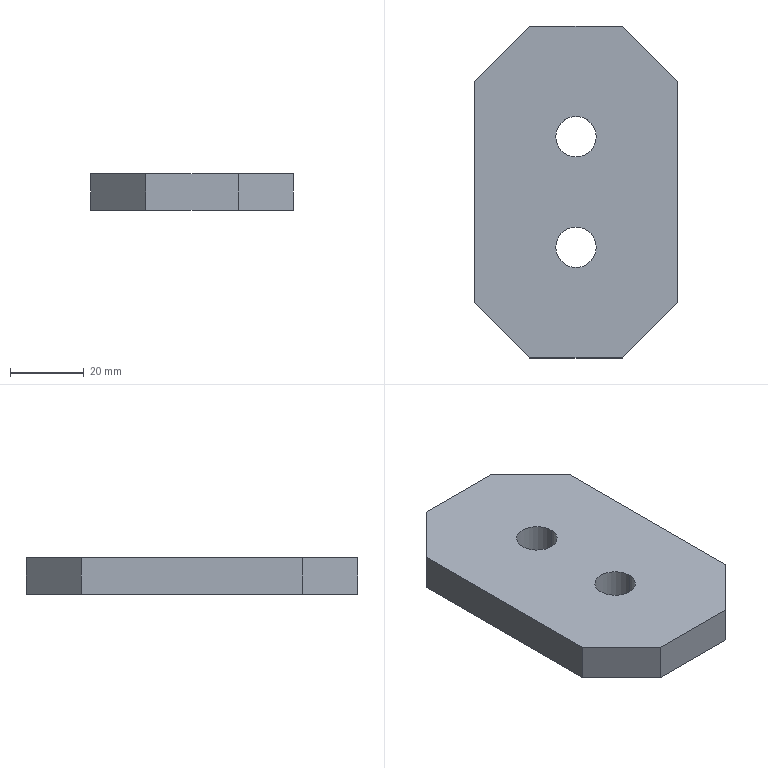Component | SolidWorks | 12ASlidingStraighteningWheelRetainingPlate-2 | 1 solid | 14 faces | box 55 x 90 x 10 mm | volume 43099 mm3 | plane 10 | cylinder 4 | commonest cylinder face diameters 11 x4 | material Q235
build123d program:
from build123d import *

# Parameters (mm, degrees)
BOSS_EXTRUDE1_DEPTH        = 10
F_11_0_11_DIAMETER_HOLE1_D = 11


with BuildPart() as part:
    # Sketch1 → Boss-Extrude1 (new body)
    with BuildSketch(Plane.XY):
        Polygon((-12.5, 45), (12.5, 45), (27.5, 30), (27.5, -30), (12.5, -45), (-12.5, -45), (-27.5, -30), (-27.5, 30), align=None)
    extrude(amount=BOSS_EXTRUDE1_DEPTH)

    # 11.0 _11_ Diameter Hole1 (through all)
    with Locations(Plane.XY.offset(10)):
        with Locations((0, -15), (0, 15)):
            Hole(F_11_0_11_DIAMETER_HOLE1_D / 2)


solid = part.part

# Placed as in the assembly
solid = solid.moved(Location((-213.402, 137.728, -24.25), (0, 0, 0)))
STEP:
#1=CARTESIAN_POINT('',(-8.185,6.013,-0.9547));
#2=VERTEX_POINT('',#1);
#3=CARTESIAN_POINT('',(-8.618,6.013,-0.9547));
#4=VERTEX_POINT('',#3);
#5=CARTESIAN_POINT('',(-8.402,6.013,-0.9547));
#6=DIRECTION('',(0.,0.,-1.));
#7=DIRECTION('',(-1.,0.,0.));
#8=AXIS2_PLACEMENT_3D('',#5,#6,#7);
#9=CIRCLE('',#8,0.2165);
#10=EDGE_CURVE('',#2,#4,#9,.T.);
#11=ORIENTED_EDGE('',*,*,#10,.T.);
#12=CARTESIAN_POINT('',(-8.618,6.013,-0.561));
#13=VERTEX_POINT('',#12);
#14=CARTESIAN_POINT('',(-8.618,6.013,-0.561));
#15=DIRECTION('',(0.,0.,1.));
#16=VECTOR('',#15,39.37);
#17=LINE('',#14,#16);
#18=EDGE_CURVE('',#4,#13,#17,.T.);
#19=ORIENTED_EDGE('',*,*,#18,.T.);
#20=CARTESIAN_POINT('',(-8.185,6.013,-0.561));
#21=VERTEX_POINT('',#20);
#22=CARTESIAN_POINT('',(-8.402,6.013,-0.561));
#23=DIRECTION('',(0.,0.,1.));
#24=DIRECTION('',(1.,0.,0.));
#25=AXIS2_PLACEMENT_3D('',#22,#23,#24);
#26=CIRCLE('',#25,0.2165);
#27=EDGE_CURVE('',#13,#21,#26,.T.);
#28=ORIENTED_EDGE('',*,*,#27,.T.);
#29=CARTESIAN_POINT('',(-8.185,6.013,-0.561));
#30=DIRECTION('',(0.,0.,1.));
#31=VECTOR('',#30,39.37);
#32=LINE('',#29,#31);
#33=EDGE_CURVE('',#2,#21,#32,.T.);
#34=ORIENTED_EDGE('',*,*,#33,.F.);
#35=EDGE_LOOP('',(#11,#19,#28,#34));
#36=FACE_OUTER_BOUND('',#35,.T.);
#37=CARTESIAN_POINT('',(-8.402,6.013,-0.561));
#38=DIRECTION('',(0.,0.,1.));
#39=DIRECTION('',(1.,0.,0.));
#40=AXIS2_PLACEMENT_3D('',#37,#38,#39);
#41=CYLINDRICAL_SURFACE('',#40,0.2165);
#42=ADVANCED_FACE('',(#36),#41,.F.);
#43=CARTESIAN_POINT('',(-8.185,4.832,-0.9547));
#44=VERTEX_POINT('',#43);
#45=CARTESIAN_POINT('',(-8.618,4.832,-0.9547));
#46=VERTEX_POINT('',#45);
#47=CARTESIAN_POINT('',(-8.402,4.832,-0.9547));
#48=DIRECTION('',(0.,0.,-1.));
#49=DIRECTION('',(-1.,0.,0.));
#50=AXIS2_PLACEMENT_3D('',#47,#48,#49);
#51=CIRCLE('',#50,0.2165);
#52=EDGE_CURVE('',#44,#46,#51,.T.);
#53=ORIENTED_EDGE('',*,*,#52,.T.);
#54=CARTESIAN_POINT('',(-8.618,4.832,-0.561));
#55=VERTEX_POINT('',#54);
#56=CARTESIAN_POINT('',(-8.618,4.832,-0.561));
#57=DIRECTION('',(0.,0.,1.));
#58=VECTOR('',#57,39.37);
#59=LINE('',#56,#58);
#60=EDGE_CURVE('',#46,#55,#59,.T.);
#61=ORIENTED_EDGE('',*,*,#60,.T.);
#62=CARTESIAN_POINT('',(-8.185,4.832,-0.561));
#63=VERTEX_POINT('',#62);
#64=CARTESIAN_POINT('',(-8.402,4.832,-0.561));
#65=DIRECTION('',(0.,0.,1.));
#66=DIRECTION('',(1.,0.,0.));
#67=AXIS2_PLACEMENT_3D('',#64,#65,#66);
#68=CIRCLE('',#67,0.2165);
#69=EDGE_CURVE('',#55,#63,#68,.T.);
#70=ORIENTED_EDGE('',*,*,#69,.T.);
#71=CARTESIAN_POINT('',(-8.185,4.832,-0.561));
#72=DIRECTION('',(0.,0.,1.));
#73=VECTOR('',#72,39.37);
#74=LINE('',#71,#73);
#75=EDGE_CURVE('',#44,#63,#74,.T.);
#76=ORIENTED_EDGE('',*,*,#75,.F.);
#77=EDGE_LOOP('',(#53,#61,#70,#76));
#78=FACE_OUTER_BOUND('',#77,.T.);
#79=CARTESIAN_POINT('',(-8.402,4.832,-0.561));
#80=DIRECTION('',(0.,0.,1.));
#81=DIRECTION('',(1.,0.,0.));
#82=AXIS2_PLACEMENT_3D('',#79,#80,#81);
#83=CYLINDRICAL_SURFACE('',#82,0.2165);
#84=ADVANCED_FACE('',(#78),#83,.F.);
#85=CARTESIAN_POINT('',(-8.402,4.832,-0.561));
#86=DIRECTION('',(0.,0.,1.));
#87=DIRECTION('',(1.,0.,0.));
#88=AXIS2_PLACEMENT_3D('',#85,#86,#87);
#89=CIRCLE('',#88,0.2165);
#90=EDGE_CURVE('',#63,#55,#89,.T.);
#91=ORIENTED_EDGE('',*,*,#90,.F.);
#92=ORIENTED_EDGE('',*,*,#69,.F.);
#93=EDGE_LOOP('',(#91,#92));
#94=FACE_BOUND('',#93,.T.);
#95=CARTESIAN_POINT('',(-8.894,7.194,-0.561));
#96=VERTEX_POINT('',#95);
#97=CARTESIAN_POINT('',(-9.484,6.603,-0.561));
#98=VERTEX_POINT('',#97);
#99=CARTESIAN_POINT('',(-9.484,6.603,-0.561));
#100=DIRECTION('',(-0.7071,-0.7071,0.));
#101=VECTOR('',#100,39.37);
#102=LINE('',#99,#101);
#103=EDGE_CURVE('',#96,#98,#102,.T.);
#104=ORIENTED_EDGE('',*,*,#103,.T.);
#105=CARTESIAN_POINT('',(-9.484,4.241,-0.561));
#106=VERTEX_POINT('',#105);
#107=CARTESIAN_POINT('',(-9.484,6.603,-0.561));
#108=DIRECTION('',(0.,-1.,0.));
#109=VECTOR('',#108,39.37);
#110=LINE('',#107,#109);
#111=EDGE_CURVE('',#98,#106,#110,.T.);
#112=ORIENTED_EDGE('',*,*,#111,.T.);
#113=CARTESIAN_POINT('',(-8.894,3.651,-0.561));
#114=VERTEX_POINT('',#113);
#115=CARTESIAN_POINT('',(-9.484,4.241,-0.561));
#116=DIRECTION('',(0.7071,-0.7071,0.));
#117=VECTOR('',#116,39.37);
#118=LINE('',#115,#117);
#119=EDGE_CURVE('',#106,#114,#118,.T.);
#120=ORIENTED_EDGE('',*,*,#119,.T.);
#121=CARTESIAN_POINT('',(-7.91,3.651,-0.561));
#122=VERTEX_POINT('',#121);
#123=CARTESIAN_POINT('',(-8.894,3.651,-0.561));
#124=DIRECTION('',(1.,0.,0.));
#125=VECTOR('',#124,39.37);
#126=LINE('',#123,#125);
#127=EDGE_CURVE('',#114,#122,#126,.T.);
#128=ORIENTED_EDGE('',*,*,#127,.T.);
#129=CARTESIAN_POINT('',(-7.319,4.241,-0.561));
#130=VERTEX_POINT('',#129);
#131=CARTESIAN_POINT('',(-7.319,4.241,-0.561));
#132=DIRECTION('',(0.7071,0.7071,0.));
#133=VECTOR('',#132,39.37);
#134=LINE('',#131,#133);
#135=EDGE_CURVE('',#122,#130,#134,.T.);
#136=ORIENTED_EDGE('',*,*,#135,.T.);
#137=CARTESIAN_POINT('',(-7.319,6.603,-0.561));
#138=VERTEX_POINT('',#137);
#139=CARTESIAN_POINT('',(-7.319,6.603,-0.561));
#140=DIRECTION('',(-0.,1.,0.));
#141=VECTOR('',#140,39.37);
#142=LINE('',#139,#141);
#143=EDGE_CURVE('',#130,#138,#142,.T.);
#144=ORIENTED_EDGE('',*,*,#143,.T.);
#145=CARTESIAN_POINT('',(-7.91,7.194,-0.561));
#146=VERTEX_POINT('',#145);
#147=CARTESIAN_POINT('',(-7.91,7.194,-0.561));
#148=DIRECTION('',(-0.7071,0.7071,0.));
#149=VECTOR('',#148,39.37);
#150=LINE('',#147,#149);
#151=EDGE_CURVE('',#138,#146,#150,.T.);
#152=ORIENTED_EDGE('',*,*,#151,.T.);
#153=CARTESIAN_POINT('',(-8.894,7.194,-0.561));
#154=DIRECTION('',(-1.,0.,0.));
#155=VECTOR('',#154,39.37);
#156=LINE('',#153,#155);
#157=EDGE_CURVE('',#146,#96,#156,.T.);
#158=ORIENTED_EDGE('',*,*,#157,.T.);
#159=EDGE_LOOP('',(#104,#112,#120,#128,#136,#144,#152,#158));
#160=FACE_OUTER_BOUND('',#159,.T.);
#161=CARTESIAN_POINT('',(-8.402,6.013,-0.561));
#162=DIRECTION('',(0.,0.,1.));
#163=DIRECTION('',(1.,0.,0.));
#164=AXIS2_PLACEMENT_3D('',#161,#162,#163);
#165=CIRCLE('',#164,0.2165);
#166=EDGE_CURVE('',#21,#13,#165,.T.);
#167=ORIENTED_EDGE('',*,*,#166,.F.);
#168=ORIENTED_EDGE('',*,*,#27,.F.);
#169=EDGE_LOOP('',(#167,#168));
#170=FACE_BOUND('',#169,.T.);
#171=CARTESIAN_POINT('',(-8.402,5.422,-0.561));
#172=DIRECTION('',(0.,0.,-1.));
#173=DIRECTION('',(-1.,0.,0.));
#174=AXIS2_PLACEMENT_3D('',#171,#172,#173);
#175=PLANE('',#174);
#176=ADVANCED_FACE('',(#94,#160,#170),#175,.F.);
#177=CARTESIAN_POINT('',(-8.894,7.194,-0.9547));
#178=VERTEX_POINT('',#177);
#179=CARTESIAN_POINT('',(-9.484,6.603,-0.9547));
#180=VERTEX_POINT('',#179);
#181=CARTESIAN_POINT('',(-9.484,6.603,-0.9547));
#182=DIRECTION('',(-0.7071,-0.7071,0.));
#183=VECTOR('',#182,39.37);
#184=LINE('',#181,#183);
#185=EDGE_CURVE('',#178,#180,#184,.T.);
#186=ORIENTED_EDGE('',*,*,#185,.T.);
#187=CARTESIAN_POINT('',(-9.484,6.603,-0.561));
#188=DIRECTION('',(0.,0.,-1.));
#189=VECTOR('',#188,39.37);
#190=LINE('',#187,#189);
#191=EDGE_CURVE('',#98,#180,#190,.T.);
#192=ORIENTED_EDGE('',*,*,#191,.F.);
#193=ORIENTED_EDGE('',*,*,#103,.F.);
#194=CARTESIAN_POINT('',(-8.894,7.194,-0.561));
#195=DIRECTION('',(0.,0.,-1.));
#196=VECTOR('',#195,39.37);
#197=LINE('',#194,#196);
#198=EDGE_CURVE('',#96,#178,#197,.T.);
#199=ORIENTED_EDGE('',*,*,#198,.T.);
#200=EDGE_LOOP('',(#186,#192,#193,#199));
#201=FACE_OUTER_BOUND('',#200,.T.);
#202=CARTESIAN_POINT('',(-9.484,6.603,-0.561));
#203=DIRECTION('',(0.7071,-0.7071,0.));
#204=DIRECTION('',(0.7071,0.7071,0.));
#205=AXIS2_PLACEMENT_3D('',#202,#203,#204);
#206=PLANE('',#205);
#207=ADVANCED_FACE('',(#201),#206,.F.);
#208=CARTESIAN_POINT('',(-9.484,4.241,-0.9547));
#209=VERTEX_POINT('',#208);
#210=CARTESIAN_POINT('',(-9.484,6.603,-0.9547));
#211=DIRECTION('',(0.,-1.,0.));
#212=VECTOR('',#211,39.37);
#213=LINE('',#210,#212);
#214=EDGE_CURVE('',#180,#209,#213,.T.);
#215=ORIENTED_EDGE('',*,*,#214,.T.);
#216=CARTESIAN_POINT('',(-9.484,4.241,-0.561));
#217=DIRECTION('',(0.,0.,-1.));
#218=VECTOR('',#217,39.37);
#219=LINE('',#216,#218);
#220=EDGE_CURVE('',#106,#209,#219,.T.);
#221=ORIENTED_EDGE('',*,*,#220,.F.);
#222=ORIENTED_EDGE('',*,*,#111,.F.);
#223=ORIENTED_EDGE('',*,*,#191,.T.);
#224=EDGE_LOOP('',(#215,#221,#222,#223));
#225=FACE_OUTER_BOUND('',#224,.T.);
#226=CARTESIAN_POINT('',(-9.484,6.603,-0.561));
#227=DIRECTION('',(1.,0.,0.));
#228=DIRECTION('',(-0.,1.,0.));
#229=AXIS2_PLACEMENT_3D('',#226,#227,#228);
#230=PLANE('',#229);
#231=ADVANCED_FACE('',(#225),#230,.F.);
#232=CARTESIAN_POINT('',(-8.894,3.651,-0.9547));
#233=VERTEX_POINT('',#232);
#234=CARTESIAN_POINT('',(-9.484,4.241,-0.9547));
#235=DIRECTION('',(0.7071,-0.7071,0.));
#236=VECTOR('',#235,39.37);
#237=LINE('',#234,#236);
#238=EDGE_CURVE('',#209,#233,#237,.T.);
#239=ORIENTED_EDGE('',*,*,#238,.T.);
#240=CARTESIAN_POINT('',(-8.894,3.651,-0.561));
#241=DIRECTION('',(0.,0.,-1.));
#242=VECTOR('',#241,39.37);
#243=LINE('',#240,#242);
#244=EDGE_CURVE('',#114,#233,#243,.T.);
#245=ORIENTED_EDGE('',*,*,#244,.F.);
#246=ORIENTED_EDGE('',*,*,#119,.F.);
#247=ORIENTED_EDGE('',*,*,#220,.T.);
#248=EDGE_LOOP('',(#239,#245,#246,#247));
#249=FACE_OUTER_BOUND('',#248,.T.);
#250=CARTESIAN_POINT('',(-9.484,4.241,-0.561));
#251=DIRECTION('',(0.7071,0.7071,0.));
#252=DIRECTION('',(-0.7071,0.7071,0.));
#253=AXIS2_PLACEMENT_3D('',#250,#251,#252);
#254=PLANE('',#253);
#255=ADVANCED_FACE('',(#249),#254,.F.);
#256=CARTESIAN_POINT('',(-7.91,3.651,-0.9547));
#257=VERTEX_POINT('',#256);
#258=CARTESIAN_POINT('',(-8.894,3.651,-0.9547));
#259=DIRECTION('',(1.,0.,0.));
#260=VECTOR('',#259,39.37);
#261=LINE('',#258,#260);
#262=EDGE_CURVE('',#233,#257,#261,.T.);
#263=ORIENTED_EDGE('',*,*,#262,.T.);
#264=CARTESIAN_POINT('',(-7.91,3.651,-0.561));
#265=DIRECTION('',(0.,0.,-1.));
#266=VECTOR('',#265,39.37);
#267=LINE('',#264,#266);
#268=EDGE_CURVE('',#122,#257,#267,.T.);
#269=ORIENTED_EDGE('',*,*,#268,.F.);
#270=ORIENTED_EDGE('',*,*,#127,.F.);
#271=ORIENTED_EDGE('',*,*,#244,.T.);
#272=EDGE_LOOP('',(#263,#269,#270,#271));
#273=FACE_OUTER_BOUND('',#272,.T.);
#274=CARTESIAN_POINT('',(-8.894,3.651,-0.561));
#275=DIRECTION('',(0.,1.,0.));
#276=DIRECTION('',(0.,0.,1.));
#277=AXIS2_PLACEMENT_3D('',#274,#275,#276);
#278=PLANE('',#277);
#279=ADVANCED_FACE('',(#273),#278,.F.);
#280=CARTESIAN_POINT('',(-7.319,4.241,-0.9547));
#281=VERTEX_POINT('',#280);
#282=CARTESIAN_POINT('',(-7.319,4.241,-0.9547));
#283=DIRECTION('',(0.7071,0.7071,0.));
#284=VECTOR('',#283,39.37);
#285=LINE('',#282,#284);
#286=EDGE_CURVE('',#257,#281,#285,.T.);
#287=ORIENTED_EDGE('',*,*,#286,.T.);
#288=CARTESIAN_POINT('',(-7.319,4.241,-0.561));
#289=DIRECTION('',(0.,0.,-1.));
#290=VECTOR('',#289,39.37);
#291=LINE('',#288,#290);
#292=EDGE_CURVE('',#130,#281,#291,.T.);
#293=ORIENTED_EDGE('',*,*,#292,.F.);
#294=ORIENTED_EDGE('',*,*,#135,.F.);
#295=ORIENTED_EDGE('',*,*,#268,.T.);
#296=EDGE_LOOP('',(#287,#293,#294,#295));
#297=FACE_OUTER_BOUND('',#296,.T.);
#298=CARTESIAN_POINT('',(-7.319,4.241,-0.561));
#299=DIRECTION('',(-0.7071,0.7071,0.));
#300=DIRECTION('',(-0.7071,-0.7071,0.));
#301=AXIS2_PLACEMENT_3D('',#298,#299,#300);
#302=PLANE('',#301);
#303=ADVANCED_FACE('',(#297),#302,.F.);
#304=CARTESIAN_POINT('',(-7.319,6.603,-0.9547));
#305=VERTEX_POINT('',#304);
#306=CARTESIAN_POINT('',(-7.319,6.603,-0.9547));
#307=DIRECTION('',(-0.,1.,0.));
#308=VECTOR('',#307,39.37);
#309=LINE('',#306,#308);
#310=EDGE_CURVE('',#281,#305,#309,.T.);
#311=ORIENTED_EDGE('',*,*,#310,.T.);
#312=CARTESIAN_POINT('',(-7.319,6.603,-0.561));
#313=DIRECTION('',(0.,0.,-1.));
#314=VECTOR('',#313,39.37);
#315=LINE('',#312,#314);
#316=EDGE_CURVE('',#138,#305,#315,.T.);
#317=ORIENTED_EDGE('',*,*,#316,.F.);
#318=ORIENTED_EDGE('',*,*,#143,.F.);
#319=ORIENTED_EDGE('',*,*,#292,.T.);
#320=EDGE_LOOP('',(#311,#317,#318,#319));
#321=FACE_OUTER_BOUND('',#320,.T.);
#322=CARTESIAN_POINT('',(-7.319,6.603,-0.561));
#323=DIRECTION('',(-1.,-0.,0.));
#324=DIRECTION('',(0.,-1.,0.));
#325=AXIS2_PLACEMENT_3D('',#322,#323,#324);
#326=PLANE('',#325);
#327=ADVANCED_FACE('',(#321),#326,.F.);
#328=CARTESIAN_POINT('',(-7.91,7.194,-0.9547));
#329=VERTEX_POINT('',#328);
#330=CARTESIAN_POINT('',(-7.91,7.194,-0.9547));
#331=DIRECTION('',(-0.7071,0.7071,0.));
#332=VECTOR('',#331,39.37);
#333=LINE('',#330,#332);
#334=EDGE_CURVE('',#305,#329,#333,.T.);
#335=ORIENTED_EDGE('',*,*,#334,.T.);
#336=CARTESIAN_POINT('',(-7.91,7.194,-0.561));
#337=DIRECTION('',(0.,0.,-1.));
#338=VECTOR('',#337,39.37);
#339=LINE('',#336,#338);
#340=EDGE_CURVE('',#146,#329,#339,.T.);
#341=ORIENTED_EDGE('',*,*,#340,.F.);
#342=ORIENTED_EDGE('',*,*,#151,.F.);
#343=ORIENTED_EDGE('',*,*,#316,.T.);
#344=EDGE_LOOP('',(#335,#341,#342,#343));
#345=FACE_OUTER_BOUND('',#344,.T.);
#346=CARTESIAN_POINT('',(-7.91,7.194,-0.561));
#347=DIRECTION('',(-0.7071,-0.7071,0.));
#348=DIRECTION('',(0.7071,-0.7071,0.));
#349=AXIS2_PLACEMENT_3D('',#346,#347,#348);
#350=PLANE('',#349);
#351=ADVANCED_FACE('',(#345),#350,.F.);
#352=CARTESIAN_POINT('',(-8.894,7.194,-0.9547));
#353=DIRECTION('',(-1.,0.,0.));
#354=VECTOR('',#353,39.37);
#355=LINE('',#352,#354);
#356=EDGE_CURVE('',#329,#178,#355,.T.);
#357=ORIENTED_EDGE('',*,*,#356,.T.);
#358=ORIENTED_EDGE('',*,*,#198,.F.);
#359=ORIENTED_EDGE('',*,*,#157,.F.);
#360=ORIENTED_EDGE('',*,*,#340,.T.);
#361=EDGE_LOOP('',(#357,#358,#359,#360));
#362=FACE_OUTER_BOUND('',#361,.T.);
#363=CARTESIAN_POINT('',(-8.894,7.194,-0.561));
#364=DIRECTION('',(0.,-1.,0.));
#365=DIRECTION('',(0.,0.,-1.));
#366=AXIS2_PLACEMENT_3D('',#363,#364,#365);
#367=PLANE('',#366);
#368=ADVANCED_FACE('',(#362),#367,.F.);
#369=ORIENTED_EDGE('',*,*,#10,.F.);
#370=CARTESIAN_POINT('',(-8.402,6.013,-0.9547));
#371=DIRECTION('',(0.,0.,-1.));
#372=DIRECTION('',(-1.,0.,0.));
#373=AXIS2_PLACEMENT_3D('',#370,#371,#372);
#374=CIRCLE('',#373,0.2165);
#375=EDGE_CURVE('',#4,#2,#374,.T.);
#376=ORIENTED_EDGE('',*,*,#375,.F.);
#377=EDGE_LOOP('',(#369,#376));
#378=FACE_BOUND('',#377,.T.);
#379=ORIENTED_EDGE('',*,*,#52,.F.);
#380=CARTESIAN_POINT('',(-8.402,4.832,-0.9547));
#381=DIRECTION('',(0.,0.,-1.));
#382=DIRECTION('',(-1.,0.,0.));
#383=AXIS2_PLACEMENT_3D('',#380,#381,#382);
#384=CIRCLE('',#383,0.2165);
#385=EDGE_CURVE('',#46,#44,#384,.T.);
#386=ORIENTED_EDGE('',*,*,#385,.F.);
#387=EDGE_LOOP('',(#379,#386));
#388=FACE_BOUND('',#387,.T.);
#389=ORIENTED_EDGE('',*,*,#185,.F.);
#390=ORIENTED_EDGE('',*,*,#356,.F.);
#391=ORIENTED_EDGE('',*,*,#334,.F.);
#392=ORIENTED_EDGE('',*,*,#310,.F.);
#393=ORIENTED_EDGE('',*,*,#286,.F.);
#394=ORIENTED_EDGE('',*,*,#262,.F.);
#395=ORIENTED_EDGE('',*,*,#238,.F.);
#396=ORIENTED_EDGE('',*,*,#214,.F.);
#397=EDGE_LOOP('',(#389,#390,#391,#392,#393,#394,#395,#396));
#398=FACE_OUTER_BOUND('',#397,.T.);
#399=CARTESIAN_POINT('',(-8.402,5.422,-0.9547));
#400=DIRECTION('',(0.,0.,-1.));
#401=DIRECTION('',(-1.,0.,0.));
#402=AXIS2_PLACEMENT_3D('',#399,#400,#401);
#403=PLANE('',#402);
#404=ADVANCED_FACE('',(#378,#388,#398),#403,.T.);
#405=ORIENTED_EDGE('',*,*,#60,.F.);
#406=ORIENTED_EDGE('',*,*,#385,.T.);
#407=ORIENTED_EDGE('',*,*,#75,.T.);
#408=ORIENTED_EDGE('',*,*,#90,.T.);
#409=EDGE_LOOP('',(#405,#406,#407,#408));
#410=FACE_OUTER_BOUND('',#409,.T.);
#411=CARTESIAN_POINT('',(-8.402,4.832,-0.561));
#412=DIRECTION('',(0.,0.,1.));
#413=DIRECTION('',(1.,0.,0.));
#414=AXIS2_PLACEMENT_3D('',#411,#412,#413);
#415=CYLINDRICAL_SURFACE('',#414,0.2165);
#416=ADVANCED_FACE('',(#410),#415,.F.);
#417=ORIENTED_EDGE('',*,*,#18,.F.);
#418=ORIENTED_EDGE('',*,*,#375,.T.);
#419=ORIENTED_EDGE('',*,*,#33,.T.);
#420=ORIENTED_EDGE('',*,*,#166,.T.);
#421=EDGE_LOOP('',(#417,#418,#419,#420));
#422=FACE_OUTER_BOUND('',#421,.T.);
#423=CARTESIAN_POINT('',(-8.402,6.013,-0.561));
#424=DIRECTION('',(0.,0.,1.));
#425=DIRECTION('',(1.,0.,0.));
#426=AXIS2_PLACEMENT_3D('',#423,#424,#425);
#427=CYLINDRICAL_SURFACE('',#426,0.2165);
#428=ADVANCED_FACE('',(#422),#427,.F.);
#429=CLOSED_SHELL('',(#42,#84,#176,#207,#231,#255,#279,#303,#327,#351,#368,#404,#416,#428));
#430=MANIFOLD_SOLID_BREP('',#429);
#431=CARTESIAN_POINT('',(0.,0.,0.));
#432=DIRECTION('',(0.,0.,1.));
#433=DIRECTION('',(1.,0.,0.));
#434=AXIS2_PLACEMENT_3D('',#431,#432,#433);
#435=(LENGTH_UNIT()NAMED_UNIT(*)SI_UNIT($,.METRE.));
#436=LENGTH_MEASURE_WITH_UNIT(LENGTH_MEASURE(0.0254),#435);
#437=DIMENSIONAL_EXPONENTS(1.,0.,0.,0.,0.,0.,0.);
#438=(CONVERSION_BASED_UNIT('',#436)LENGTH_UNIT()NAMED_UNIT(#437));
#439=UNCERTAINTY_MEASURE_WITH_UNIT(LENGTH_MEASURE(0.00001),#438,'','');
#440=(NAMED_UNIT(*)PLANE_ANGLE_UNIT()SI_UNIT($,.RADIAN.));
#441=(NAMED_UNIT(*)SI_UNIT($,.STERADIAN.)SOLID_ANGLE_UNIT());
#442=(GEOMETRIC_REPRESENTATION_CONTEXT(3)GLOBAL_UNCERTAINTY_ASSIGNED_CONTEXT((#439))GLOBAL_UNIT_ASSIGNED_CONTEXT((#438,#440,#441))REPRESENTATION_CONTEXT('',''));
#443=ADVANCED_BREP_SHAPE_REPRESENTATION('',(#430,#434),#442);
#444=COLOUR_RGB('',0.7922,0.8196,0.9333);
#445=FILL_AREA_STYLE_COLOUR('',#444);
#446=FILL_AREA_STYLE('',(#445));
#447=SURFACE_STYLE_FILL_AREA(#446);
#448=SURFACE_SIDE_STYLE('',(#447));
#449=SURFACE_STYLE_USAGE(.BOTH.,#448);
#450=PRESENTATION_STYLE_ASSIGNMENT((#449));
#451=STYLED_ITEM('',(#450),#430);
#452=PRESENTATION_LAYER_ASSIGNMENT('','',(#451));
#453=(LENGTH_UNIT()NAMED_UNIT(*)SI_UNIT($,.METRE.));
#454=LENGTH_MEASURE_WITH_UNIT(LENGTH_MEASURE(0.0254),#453);
#455=DIMENSIONAL_EXPONENTS(1.,0.,0.,0.,0.,0.,0.);
#456=(CONVERSION_BASED_UNIT('',#454)LENGTH_UNIT()NAMED_UNIT(#455));
#457=UNCERTAINTY_MEASURE_WITH_UNIT(LENGTH_MEASURE(0.00001),#456,'','');
#458=(NAMED_UNIT(*)PLANE_ANGLE_UNIT()SI_UNIT($,.RADIAN.));
#459=(NAMED_UNIT(*)SI_UNIT($,.STERADIAN.)SOLID_ANGLE_UNIT());
#460=(GEOMETRIC_REPRESENTATION_CONTEXT(3)GLOBAL_UNCERTAINTY_ASSIGNED_CONTEXT((#457))GLOBAL_UNIT_ASSIGNED_CONTEXT((#456,#458,#459))REPRESENTATION_CONTEXT('',''));
#461=MECHANICAL_DESIGN_GEOMETRIC_PRESENTATION_REPRESENTATION('',(#451),#460);